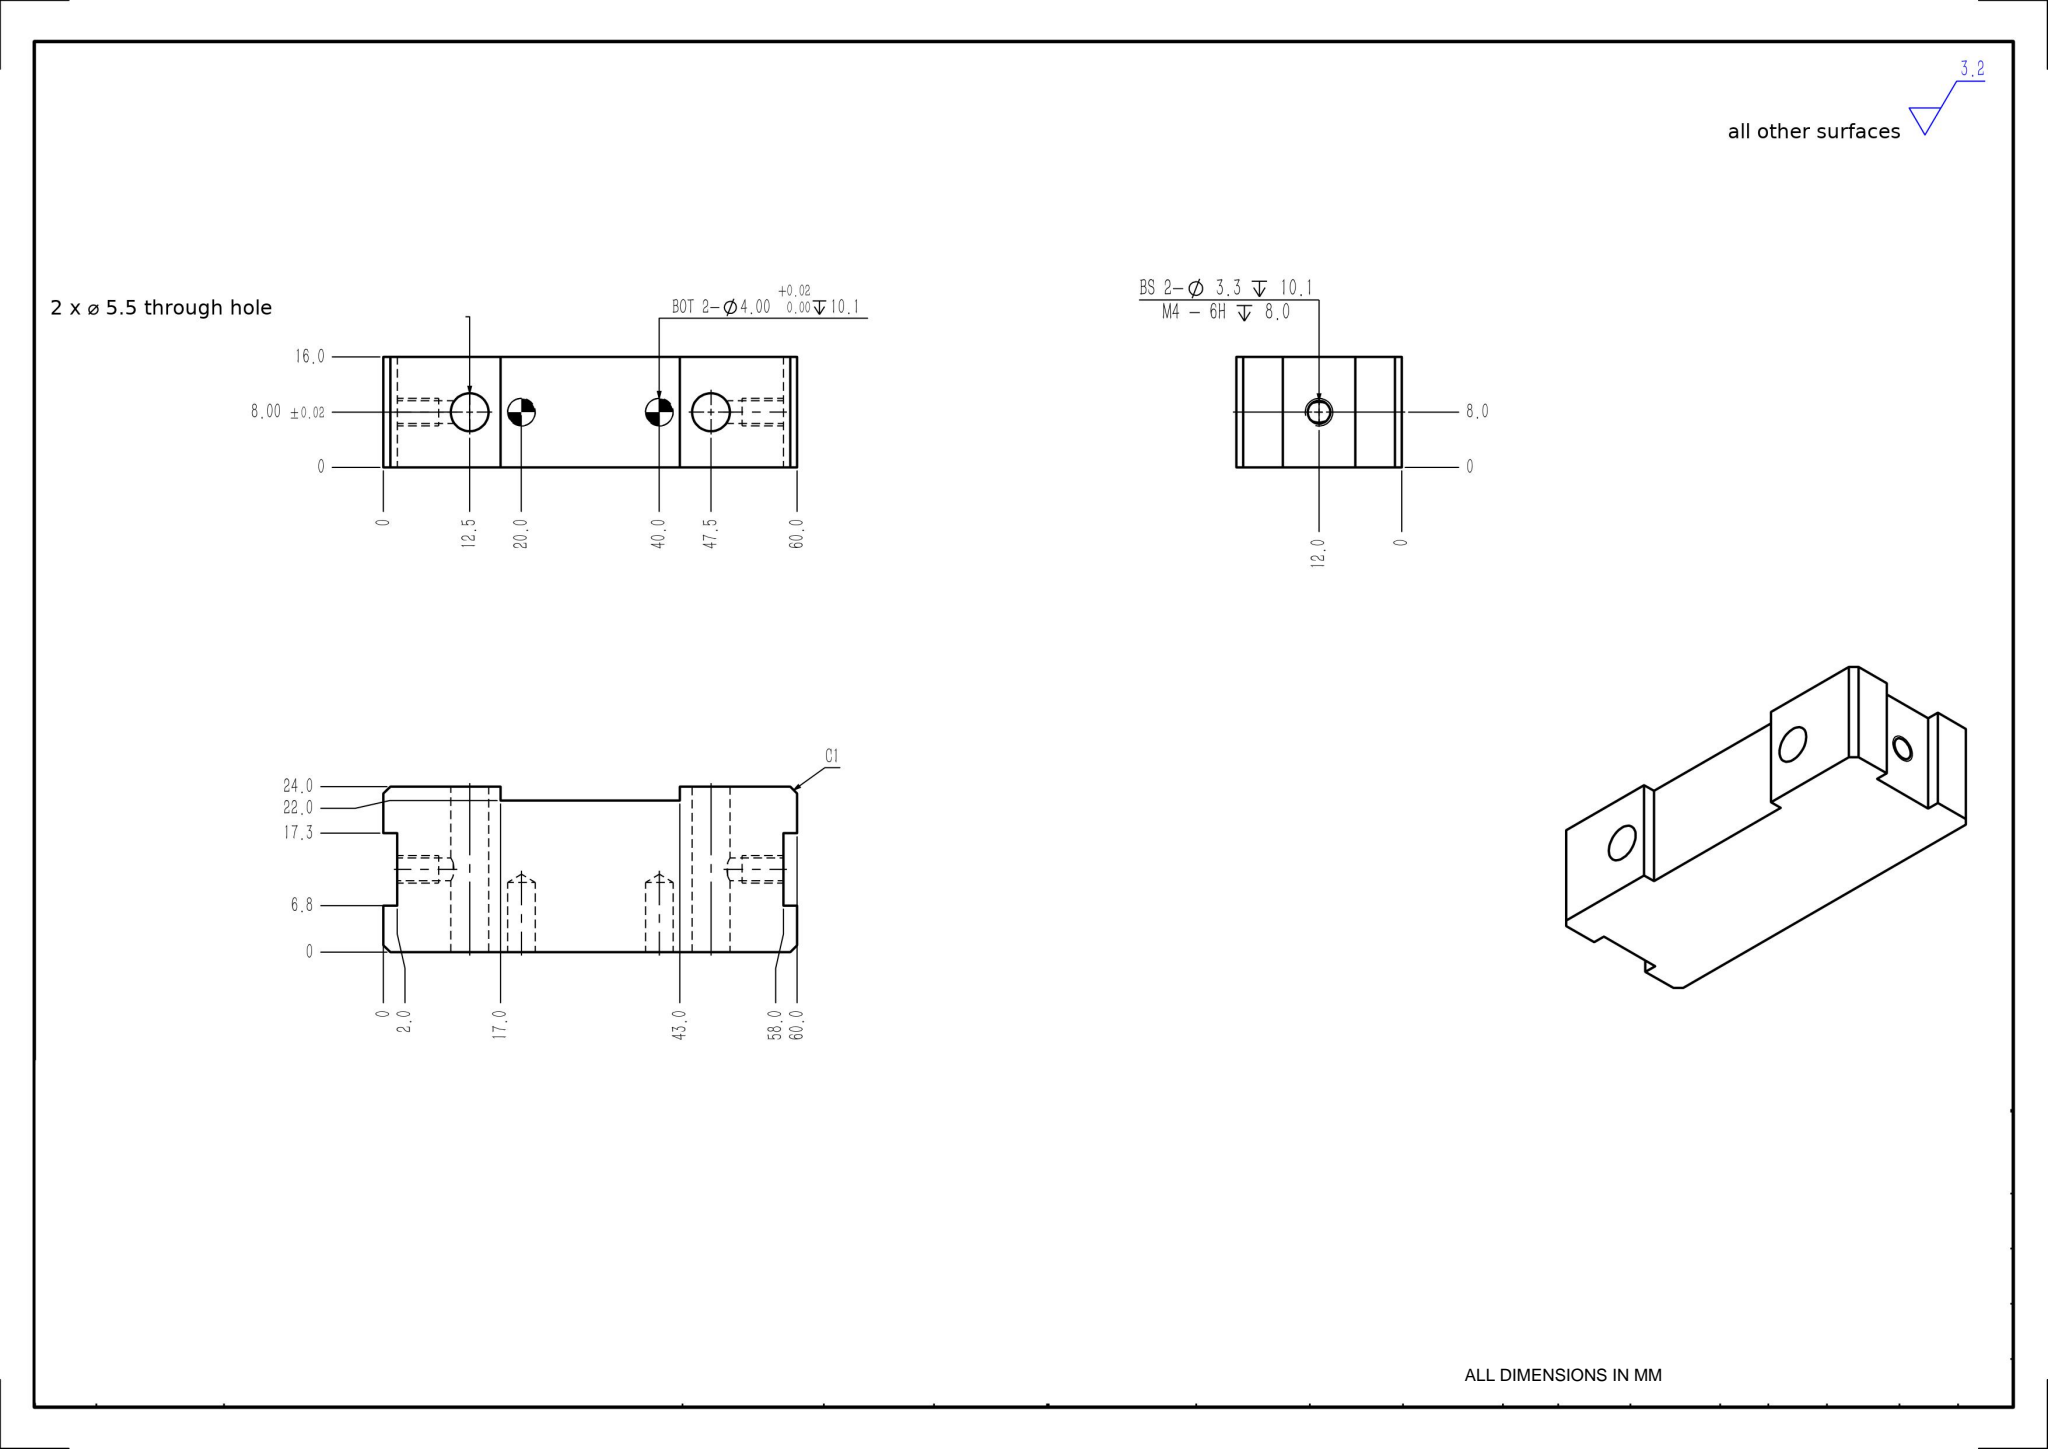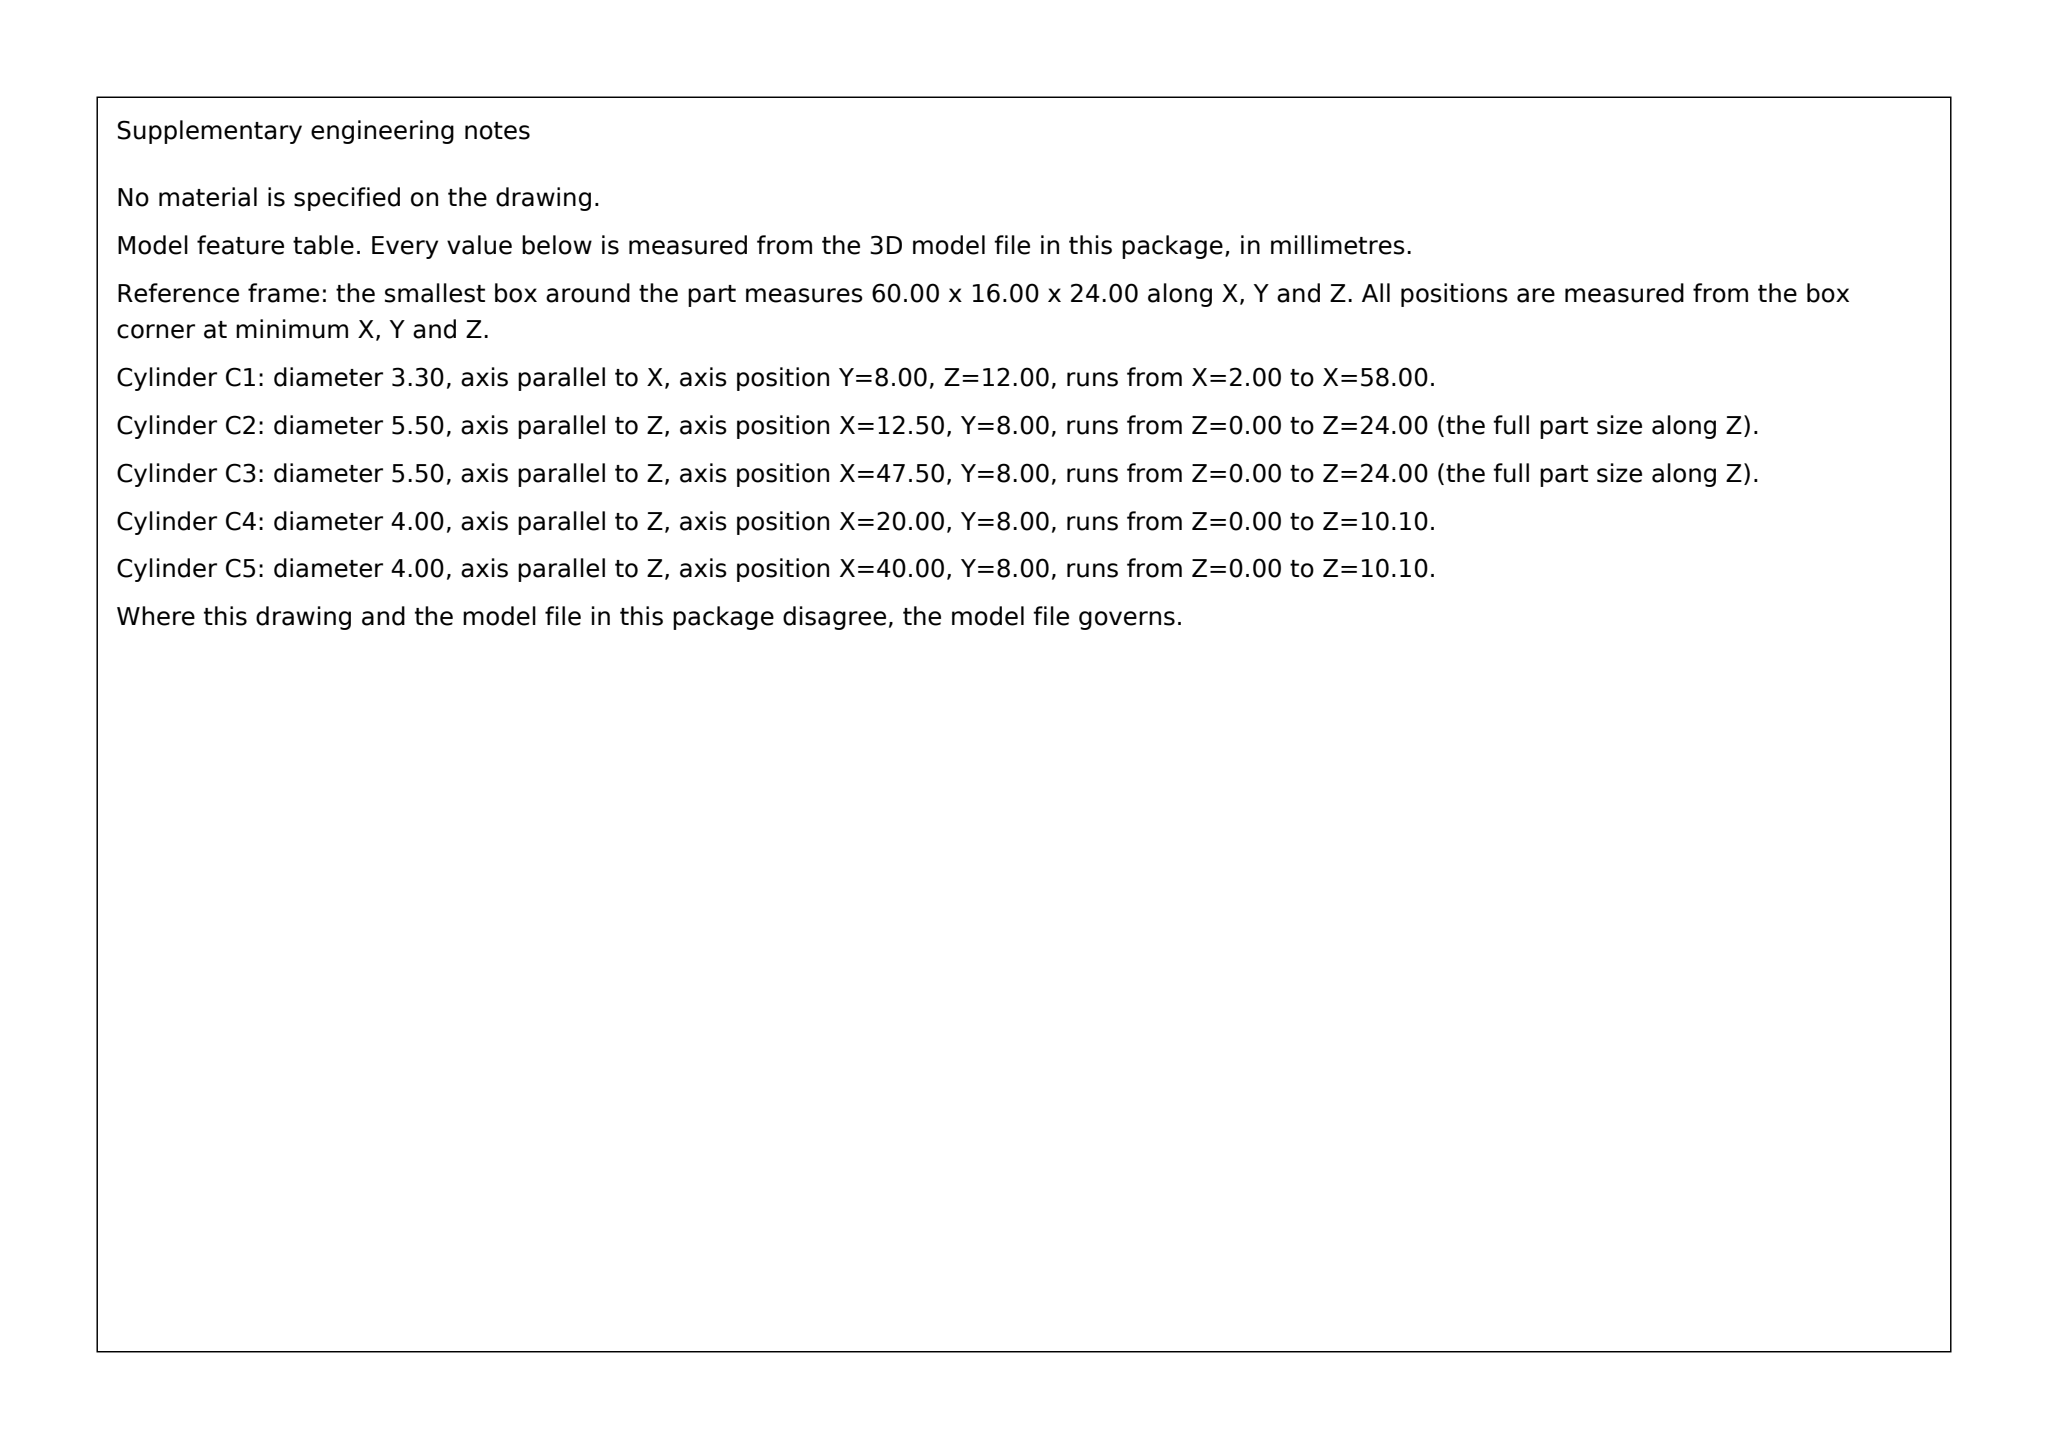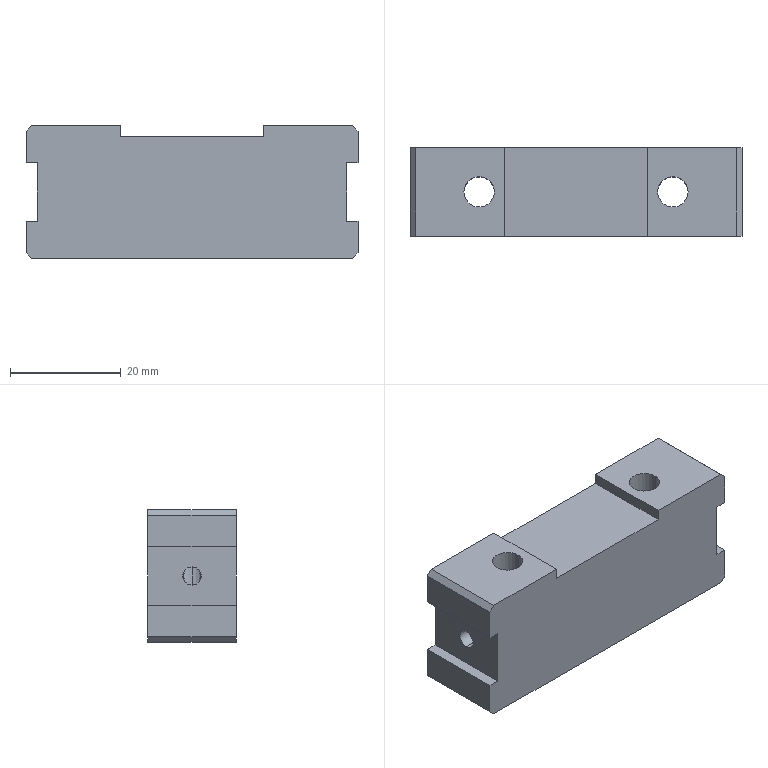Part | SolidWorks | mm | 1 solid | 42 faces | box 60 x 16 x 24 mm | volume 19965 mm3 | plane 22 | cylinder 12 | cone 8 | commonest cylinder face diameters 3.3 x4 5.5 x4 4 x4
build123d program:
from build123d import *

# Parameters (mm, degrees)
SKETCH1_W                      = 60
SKETCH1_H                      = 16
BOSS_EXTRUDE1_DEPTH            = 12
SKETCH2_W                      = 26
SKETCH2_H                      = 16
CUT_EXTRUDE1_DEPTH             = 2
SIZE_MM_DOWEL_PIN_HOLE_1_D     = 4
SIZE_MM_DOWEL_PIN_HOLE_1_DEPTH = 10.1
SIZE_MM_DOWEL_PIN_HOLE_1_TIP   = 1.202
F_5_5_5_5_DIAMETER_HOLE1_D     = 5.5
SKETCH12_W                     = 12
SKETCH12_H                     = 10.5
CUT_EXTRUDE3_DEPTH             = 37.056
M4_TAPPED_HOLE1_D              = 3.3
M4_TAPPED_HOLE1_DEPTH          = 10.1
M4_TAPPED_HOLE1_TIP            = 0.9914
M4_TAPPED_HOLE2_D              = 3.3
M4_TAPPED_HOLE2_DEPTH          = 10.1
M4_TAPPED_HOLE2_TIP            = 0.9914
CHAMFER1_SIZE                  = 1


with BuildPart() as part:
    # Sketch1 → Boss-Extrude1 (new, symmetric)
    with BuildSketch(Plane.XY):
        Rectangle(SKETCH1_W, SKETCH1_H)
    extrude(amount=BOSS_EXTRUDE1_DEPTH, both=True)

    # Sketch2 → Cut-Extrude1 (cut)
    with BuildSketch(Plane.XY.offset(12)):
        Rectangle(SKETCH2_W, SKETCH2_H)
    extrude(amount=-CUT_EXTRUDE1_DEPTH, mode=Mode.SUBTRACT)

    # Size mm Dowel Pin Hole 1
    with Locations(Plane(origin=(0, 0, -12), x_dir=(-1, 0, 0), z_dir=(0, 0, -1))):
        with Locations((-10, 0), (10, 0)):
            Hole(SIZE_MM_DOWEL_PIN_HOLE_1_D / 2, depth=SIZE_MM_DOWEL_PIN_HOLE_1_DEPTH)
            with Locations((0, 0, -(SIZE_MM_DOWEL_PIN_HOLE_1_DEPTH + SIZE_MM_DOWEL_PIN_HOLE_1_TIP / 2))):  # 118° drill point
                Cone(0, SIZE_MM_DOWEL_PIN_HOLE_1_D / 2, SIZE_MM_DOWEL_PIN_HOLE_1_TIP, mode=Mode.SUBTRACT)

    # 5.5 _5.5_ Diameter Hole1 (through all)
    with Locations(Plane.XY.offset(12)):
        with Locations((-17.5, 0), (17.5, 0)):
            Hole(F_5_5_5_5_DIAMETER_HOLE1_D / 2)

    # Sketch12 → Cut-Extrude3 (cut, through all)
    with BuildSketch(Plane(origin=(0, 8, 0), x_dir=(1, 0, 0), z_dir=(0, 1, 0))):
        with Locations((-34, 0)):
            Rectangle(SKETCH12_W, SKETCH12_H)
        with Locations((34, 0)):
            Rectangle(SKETCH12_W, SKETCH12_H)
    extrude(amount=-CUT_EXTRUDE3_DEPTH, mode=Mode.SUBTRACT)

    # M4 Tapped Hole1
    with Locations(Plane.ZY.offset(30)):
        with Locations((0, 0)):
            Hole(M4_TAPPED_HOLE1_D / 2, depth=M4_TAPPED_HOLE1_DEPTH)
            with Locations((0, 0, -(M4_TAPPED_HOLE1_DEPTH + M4_TAPPED_HOLE1_TIP / 2))):  # 118° drill point
                Cone(0, M4_TAPPED_HOLE1_D / 2, M4_TAPPED_HOLE1_TIP, mode=Mode.SUBTRACT)

    # M4 Tapped Hole2
    with Locations(Plane(origin=(30, 0, 0), x_dir=(0, 0, -1), z_dir=(1, 0, 0))):
        with Locations((0, 0)):
            Hole(M4_TAPPED_HOLE2_D / 2, depth=M4_TAPPED_HOLE2_DEPTH)
            with Locations((0, 0, -(M4_TAPPED_HOLE2_DEPTH + M4_TAPPED_HOLE2_TIP / 2))):  # 118° drill point
                Cone(0, M4_TAPPED_HOLE2_D / 2, M4_TAPPED_HOLE2_TIP, mode=Mode.SUBTRACT)

    # Chamfer1
    chamfer1_edges = [part.edges().sort_by_distance(p)[0] for p in [
        (-30, 0, 12),
        (30, 0, 12),
        (-30, 0, -12),
        (30, 0, -12),
    ]]
    chamfer(chamfer1_edges, length=CHAMFER1_SIZE)


solid = part.part